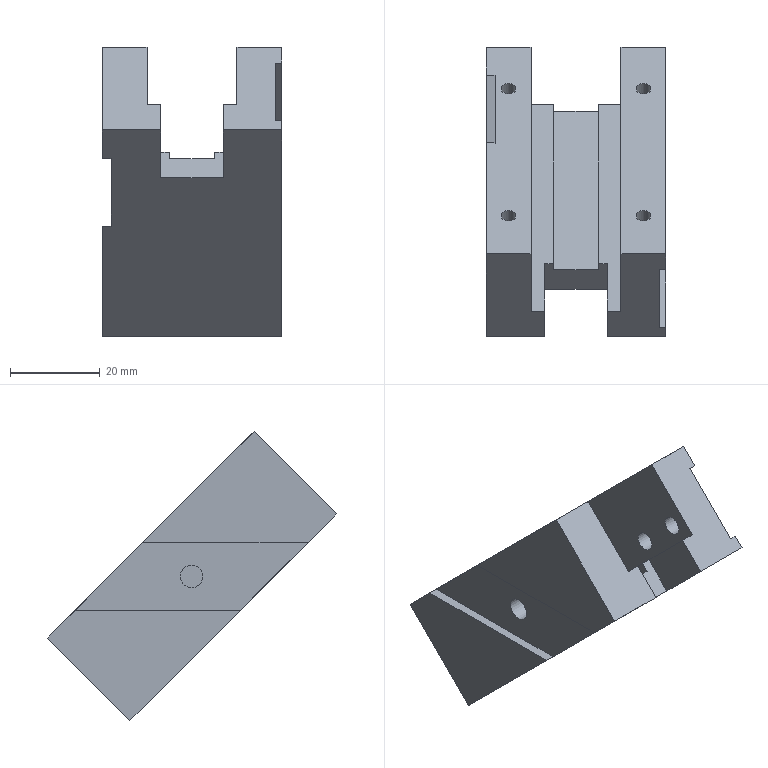Component | SolidWorks | ZL-10-03SlideChannel-1 | 1 solid | 48 faces | box 40 x 64.35 x 64.35 mm | volume 37912 mm3 | plane 26 | cylinder 14 | cone 8 | commonest cylinder face diameters 3.3 x8 4.2 x4 5 x2
build123d program:
from build123d import *

# Parameters (mm, degrees)
EXTRUDE1_DEPTH             = 65
M4_TAPPED_HOLE1_AT_2_COUNT = 2
M4_TAPPED_HOLE1_AT_2_PITCH = 40
SKETCH4_W                  = 1.5
SKETCH4_H                  = 18
CUT_EXTRUDE1_DEPTH         = 73.808
M5_TAPPED_HOLE1_D          = 4.2
M5_TAPPED_HOLE1_DEPTH      = 8.5
SKETCH8_W                  = 14
SKETCH8_H                  = 15
CUT_EXTRUDE2_DEPTH         = 71.349
SKETCH9_W                  = 10
SKETCH9_H                  = 50
CUT_EXTRUDE3_DEPTH         = 2
CUT_EXTRUDE4_DEPTH         = 2
M6_TAPPED_HOLE1_D          = 5
M6_TAPPED_HOLE1_DEPTH      = 8


with BuildPart() as part:
    # Sketch1 → Extrude1 (new body)
    with BuildSketch(Plane(origin=(0, 0, 0), x_dir=(1, 0, 0), z_dir=(0, 1, 0))):
        Polygon((20, 0), (-20, 0), (-20, 26), (-10, 26), (-10, 8), (10, 8), (10, 26), (20, 26), align=None)
    extrude(amount=EXTRUDE1_DEPTH)

    # Sketch2 → M4 Tapped Hole1 (revolve, cut)
    with BuildSketch(Plane(origin=(15, 52, -26), x_dir=(0, 1, 0), z_dir=(1, 0, 0))):
        Polygon((0, 0), (0, 11.091), (1.65, 10.1), (1.65, 0), align=None)
    m4_tapped_hole1 = revolve(axis=Axis((15, 52, -32.35), (0, 0, 1)), mode=Mode.SUBTRACT)

    # M4 Tapped Hole1 at 2: M4 Tapped Hole1 ×2
    with Locations(*[(0, -i * M4_TAPPED_HOLE1_AT_2_PITCH, 0) for i in range(1, M4_TAPPED_HOLE1_AT_2_COUNT)]):
        add(m4_tapped_hole1, mode=Mode.SUBTRACT)

    # Mirror1: M4 Tapped Hole1 across plane
    add(m4_tapped_hole1.mirror(Plane(origin=(0, 0, 0), x_dir=(0, 0, 1), z_dir=(1, 0, 0))), mode=Mode.SUBTRACT)

    # Mirror1 copy 1 sketch → Mirror1 copy 1 (revolve, cut)
    with BuildSketch(Plane(origin=(-15, 12, -26), x_dir=(0, 1, 0), z_dir=(-1, 0, 0))):
        Polygon((0, 0), (0, -11.091), (1.65, -10.1), (1.65, 0), align=None)
    revolve(axis=Axis((-15, 12, -32.35), (0, 0, -1)), mode=Mode.SUBTRACT)

    # Sketch4 → Cut-Extrude1 (cut, through all)
    with BuildSketch(Plane.XZ):
        with Locations((-19.25, -12)):
            Rectangle(SKETCH4_W, SKETCH4_H)
    extrude(amount=-CUT_EXTRUDE1_DEPTH, mode=Mode.SUBTRACT)

    # M5 Tapped Hole1
    with Locations(Plane.ZY.offset(18.5)):
        with Locations((-12, 5), (-12, 17)):
            Hole(M5_TAPPED_HOLE1_D / 2, depth=M5_TAPPED_HOLE1_DEPTH)

    # Sketch8 → Cut-Extrude2 (cut, through all)
    with BuildSketch(Plane(origin=(0, 0, -8), x_dir=(-1, 0, 0), z_dir=(0, 0, -1))):
        with Locations((0, 7.5)):
            Rectangle(SKETCH8_W, SKETCH8_H)
    extrude(amount=-CUT_EXTRUDE2_DEPTH, mode=Mode.SUBTRACT)

    # Sketch9 → Cut-Extrude3 (cut)
    with BuildSketch(Plane(origin=(0, 0, -8), x_dir=(-1, 0, 0), z_dir=(0, 0, -1))):
        with Locations((0, 40)):
            Rectangle(SKETCH9_W, SKETCH9_H)
    extrude(amount=-CUT_EXTRUDE3_DEPTH, mode=Mode.SUBTRACT)

    # Sketch10 → Cut-Extrude4 (cut)
    with BuildSketch(Plane(origin=(20, 0, 0), x_dir=(0, 0, -1), z_dir=(1, 0, 0))):
        Polygon((26, 35), (0, 9), (0, 30.213), (26, 56.213), align=None)
    extrude(amount=-CUT_EXTRUDE4_DEPTH, mode=Mode.SUBTRACT)

    # M6 Tapped Hole1
    with Locations(Plane(origin=(18, 0, 0), x_dir=(0, 0, -1), z_dir=(1, 0, 0))):
        with Locations((13, 32.607)):
            Hole(M6_TAPPED_HOLE1_D / 2, depth=M6_TAPPED_HOLE1_DEPTH)


solid = part.part

# Placed as in the assembly
solid = solid.moved(Location((42.823, 31.501, -3.136), (135, 0, 180)))